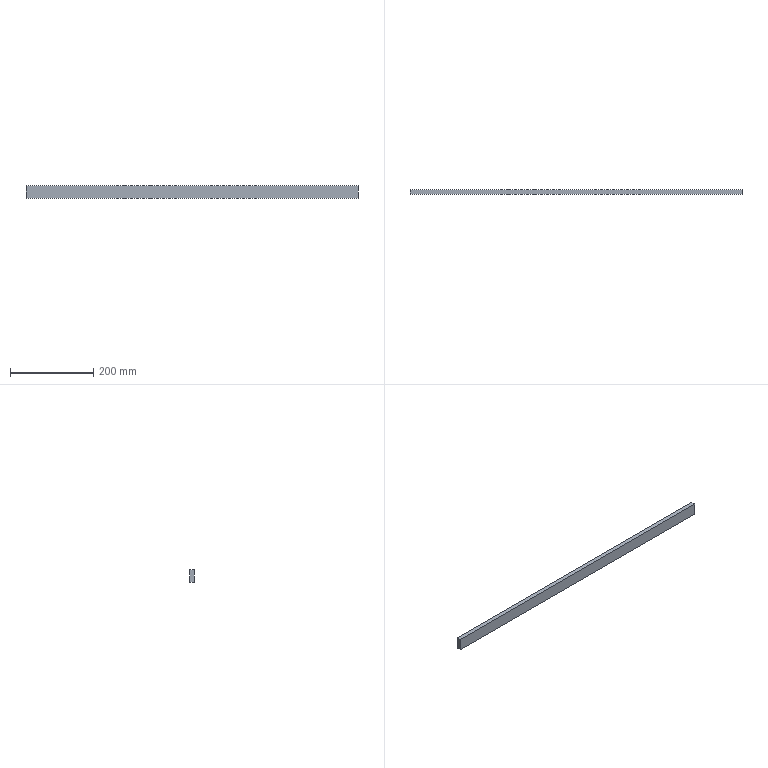Component | SolidWorks | JF21-80.1-1-3(_)-1-SOLID30-1 | 1 solid | 6 faces | box 800 x 10 x 30 mm | volume 240000 mm3 | plane 6
STEP:
#1=COLOUR_RGB('',0.7922,0.8196,0.9333);
#2=FILL_AREA_STYLE_COLOUR('',#1);
#3=FILL_AREA_STYLE('',(#2));
#4=SURFACE_STYLE_FILL_AREA(#3);
#5=SURFACE_SIDE_STYLE('',(#4));
#6=SURFACE_STYLE_USAGE(.BOTH.,#5);
#7=PRESENTATION_STYLE_ASSIGNMENT((#6));
#8=CARTESIAN_POINT('',(-15.748,15.354,23.819));
#9=VERTEX_POINT('',#8);
#10=CARTESIAN_POINT('',(-15.748,15.354,25.));
#11=VERTEX_POINT('',#10);
#12=CARTESIAN_POINT('',(-15.748,15.354,25.));
#13=DIRECTION('',(0.,0.,1.));
#14=VECTOR('',#13,39.37);
#15=LINE('',#12,#14);
#16=EDGE_CURVE('',#9,#11,#15,.T.);
#17=ORIENTED_EDGE('',*,*,#16,.F.);
#18=CARTESIAN_POINT('',(-15.748,14.961,23.819));
#19=VERTEX_POINT('',#18);
#20=CARTESIAN_POINT('',(-15.748,14.961,23.819));
#21=DIRECTION('',(-0.,1.,0.));
#22=VECTOR('',#21,39.37);
#23=LINE('',#20,#22);
#24=EDGE_CURVE('',#19,#9,#23,.T.);
#25=ORIENTED_EDGE('',*,*,#24,.F.);
#26=CARTESIAN_POINT('',(-15.748,14.961,25.));
#27=VERTEX_POINT('',#26);
#28=CARTESIAN_POINT('',(-15.748,14.961,25.));
#29=DIRECTION('',(0.,0.,1.));
#30=VECTOR('',#29,39.37);
#31=LINE('',#28,#30);
#32=EDGE_CURVE('',#19,#27,#31,.T.);
#33=ORIENTED_EDGE('',*,*,#32,.T.);
#34=CARTESIAN_POINT('',(-15.748,14.961,25.));
#35=DIRECTION('',(-0.,1.,0.));
#36=VECTOR('',#35,39.37);
#37=LINE('',#34,#36);
#38=EDGE_CURVE('',#27,#11,#37,.T.);
#39=ORIENTED_EDGE('',*,*,#38,.T.);
#40=EDGE_LOOP('',(#17,#25,#33,#39));
#41=FACE_OUTER_BOUND('',#40,.T.);
#42=CARTESIAN_POINT('',(-15.748,14.961,25.));
#43=DIRECTION('',(-1.,-0.,0.));
#44=DIRECTION('',(-0.,1.,0.));
#45=AXIS2_PLACEMENT_3D('',#42,#43,#44);
#46=PLANE('',#45);
#47=ADVANCED_FACE('',(#41),#46,.T.);
#48=CARTESIAN_POINT('',(15.748,15.354,23.819));
#49=VERTEX_POINT('',#48);
#50=CARTESIAN_POINT('',(-15.748,15.354,23.819));
#51=DIRECTION('',(-1.,-0.,0.));
#52=VECTOR('',#51,39.37);
#53=LINE('',#50,#52);
#54=EDGE_CURVE('',#49,#9,#53,.T.);
#55=ORIENTED_EDGE('',*,*,#54,.F.);
#56=CARTESIAN_POINT('',(15.748,14.961,23.819));
#57=VERTEX_POINT('',#56);
#58=CARTESIAN_POINT('',(15.748,14.961,23.819));
#59=DIRECTION('',(-0.,1.,0.));
#60=VECTOR('',#59,39.37);
#61=LINE('',#58,#60);
#62=EDGE_CURVE('',#57,#49,#61,.T.);
#63=ORIENTED_EDGE('',*,*,#62,.F.);
#64=CARTESIAN_POINT('',(-15.748,14.961,23.819));
#65=DIRECTION('',(-1.,-0.,0.));
#66=VECTOR('',#65,39.37);
#67=LINE('',#64,#66);
#68=EDGE_CURVE('',#57,#19,#67,.T.);
#69=ORIENTED_EDGE('',*,*,#68,.T.);
#70=ORIENTED_EDGE('',*,*,#24,.T.);
#71=EDGE_LOOP('',(#55,#63,#69,#70));
#72=FACE_OUTER_BOUND('',#71,.T.);
#73=CARTESIAN_POINT('',(-15.748,14.961,23.819));
#74=DIRECTION('',(-0.,-0.,-1.));
#75=DIRECTION('',(1.,0.,-0.));
#76=AXIS2_PLACEMENT_3D('',#73,#74,#75);
#77=PLANE('',#76);
#78=ADVANCED_FACE('',(#72),#77,.T.);
#79=CARTESIAN_POINT('',(15.748,15.354,25.));
#80=VERTEX_POINT('',#79);
#81=CARTESIAN_POINT('',(15.748,15.354,25.));
#82=DIRECTION('',(0.,0.,-1.));
#83=VECTOR('',#82,39.37);
#84=LINE('',#81,#83);
#85=EDGE_CURVE('',#80,#49,#84,.T.);
#86=ORIENTED_EDGE('',*,*,#85,.F.);
#87=CARTESIAN_POINT('',(15.748,14.961,25.));
#88=VERTEX_POINT('',#87);
#89=CARTESIAN_POINT('',(15.748,14.961,25.));
#90=DIRECTION('',(-0.,1.,0.));
#91=VECTOR('',#90,39.37);
#92=LINE('',#89,#91);
#93=EDGE_CURVE('',#88,#80,#92,.T.);
#94=ORIENTED_EDGE('',*,*,#93,.F.);
#95=CARTESIAN_POINT('',(15.748,14.961,25.));
#96=DIRECTION('',(0.,0.,-1.));
#97=VECTOR('',#96,39.37);
#98=LINE('',#95,#97);
#99=EDGE_CURVE('',#88,#57,#98,.T.);
#100=ORIENTED_EDGE('',*,*,#99,.T.);
#101=ORIENTED_EDGE('',*,*,#62,.T.);
#102=EDGE_LOOP('',(#86,#94,#100,#101));
#103=FACE_OUTER_BOUND('',#102,.T.);
#104=CARTESIAN_POINT('',(15.748,14.961,25.));
#105=DIRECTION('',(1.,0.,0.));
#106=DIRECTION('',(0.,-1.,0.));
#107=AXIS2_PLACEMENT_3D('',#104,#105,#106);
#108=PLANE('',#107);
#109=ADVANCED_FACE('',(#103),#108,.T.);
#110=CARTESIAN_POINT('',(-15.748,15.354,25.));
#111=DIRECTION('',(1.,0.,-0.));
#112=VECTOR('',#111,39.37);
#113=LINE('',#110,#112);
#114=EDGE_CURVE('',#11,#80,#113,.T.);
#115=ORIENTED_EDGE('',*,*,#114,.F.);
#116=ORIENTED_EDGE('',*,*,#38,.F.);
#117=CARTESIAN_POINT('',(-15.748,14.961,25.));
#118=DIRECTION('',(1.,0.,-0.));
#119=VECTOR('',#118,39.37);
#120=LINE('',#117,#119);
#121=EDGE_CURVE('',#27,#88,#120,.T.);
#122=ORIENTED_EDGE('',*,*,#121,.T.);
#123=ORIENTED_EDGE('',*,*,#93,.T.);
#124=EDGE_LOOP('',(#115,#116,#122,#123));
#125=FACE_OUTER_BOUND('',#124,.T.);
#126=CARTESIAN_POINT('',(-15.748,14.961,25.));
#127=DIRECTION('',(0.,0.,1.));
#128=DIRECTION('',(-1.,0.,0.));
#129=AXIS2_PLACEMENT_3D('',#126,#127,#128);
#130=PLANE('',#129);
#131=ADVANCED_FACE('',(#125),#130,.T.);
#132=ORIENTED_EDGE('',*,*,#32,.F.);
#133=ORIENTED_EDGE('',*,*,#68,.F.);
#134=ORIENTED_EDGE('',*,*,#99,.F.);
#135=ORIENTED_EDGE('',*,*,#121,.F.);
#136=EDGE_LOOP('',(#132,#133,#134,#135));
#137=FACE_OUTER_BOUND('',#136,.T.);
#138=CARTESIAN_POINT('',(-15.748,14.961,23.819));
#139=DIRECTION('',(0.,-1.,0.));
#140=DIRECTION('',(-1.,-0.,0.));
#141=AXIS2_PLACEMENT_3D('',#138,#139,#140);
#142=PLANE('',#141);
#143=ADVANCED_FACE('',(#137),#142,.T.);
#144=ORIENTED_EDGE('',*,*,#16,.T.);
#145=ORIENTED_EDGE('',*,*,#114,.T.);
#146=ORIENTED_EDGE('',*,*,#85,.T.);
#147=ORIENTED_EDGE('',*,*,#54,.T.);
#148=EDGE_LOOP('',(#144,#145,#146,#147));
#149=FACE_OUTER_BOUND('',#148,.T.);
#150=CARTESIAN_POINT('',(-15.748,15.354,23.819));
#151=DIRECTION('',(0.,-1.,0.));
#152=DIRECTION('',(-1.,-0.,0.));
#153=AXIS2_PLACEMENT_3D('',#150,#151,#152);
#154=PLANE('',#153);
#155=ADVANCED_FACE('',(#149),#154,.F.);
#156=CLOSED_SHELL('',(#47,#78,#109,#131,#143,#155));
#157=MANIFOLD_SOLID_BREP('',#156);
#158=STYLED_ITEM('',(#7),#157);
#159=PRESENTATION_LAYER_ASSIGNMENT('','',(#158));
#160=(LENGTH_UNIT()NAMED_UNIT(*)SI_UNIT($,.METRE.));
#161=LENGTH_MEASURE_WITH_UNIT(LENGTH_MEASURE(0.0254),#160);
#162=DIMENSIONAL_EXPONENTS(1.,0.,0.,0.,0.,0.,0.);
#163=(CONVERSION_BASED_UNIT('',#161)LENGTH_UNIT()NAMED_UNIT(#162));
#164=UNCERTAINTY_MEASURE_WITH_UNIT(LENGTH_MEASURE(0.00001),#163,'','');
#165=(NAMED_UNIT(*)PLANE_ANGLE_UNIT()SI_UNIT($,.RADIAN.));
#166=(NAMED_UNIT(*)SI_UNIT($,.STERADIAN.)SOLID_ANGLE_UNIT());
#167=(GEOMETRIC_REPRESENTATION_CONTEXT(3)GLOBAL_UNCERTAINTY_ASSIGNED_CONTEXT((#164))GLOBAL_UNIT_ASSIGNED_CONTEXT((#163,#165,#166))REPRESENTATION_CONTEXT('',''));
#168=MECHANICAL_DESIGN_GEOMETRIC_PRESENTATION_REPRESENTATION('',(#158),#167);
#169=CARTESIAN_POINT('',(0.,0.,0.));
#170=DIRECTION('',(0.,0.,1.));
#171=DIRECTION('',(1.,0.,0.));
#172=AXIS2_PLACEMENT_3D('',#169,#170,#171);
#173=(LENGTH_UNIT()NAMED_UNIT(*)SI_UNIT($,.METRE.));
#174=LENGTH_MEASURE_WITH_UNIT(LENGTH_MEASURE(0.0254),#173);
#175=DIMENSIONAL_EXPONENTS(1.,0.,0.,0.,0.,0.,0.);
#176=(CONVERSION_BASED_UNIT('',#174)LENGTH_UNIT()NAMED_UNIT(#175));
#177=UNCERTAINTY_MEASURE_WITH_UNIT(LENGTH_MEASURE(0.00001),#176,'','');
#178=(NAMED_UNIT(*)PLANE_ANGLE_UNIT()SI_UNIT($,.RADIAN.));
#179=(NAMED_UNIT(*)SI_UNIT($,.STERADIAN.)SOLID_ANGLE_UNIT());
#180=(GEOMETRIC_REPRESENTATION_CONTEXT(3)GLOBAL_UNCERTAINTY_ASSIGNED_CONTEXT((#177))GLOBAL_UNIT_ASSIGNED_CONTEXT((#176,#178,#179))REPRESENTATION_CONTEXT('',''));
#181=ADVANCED_BREP_SHAPE_REPRESENTATION('',(#157,#172),#180);